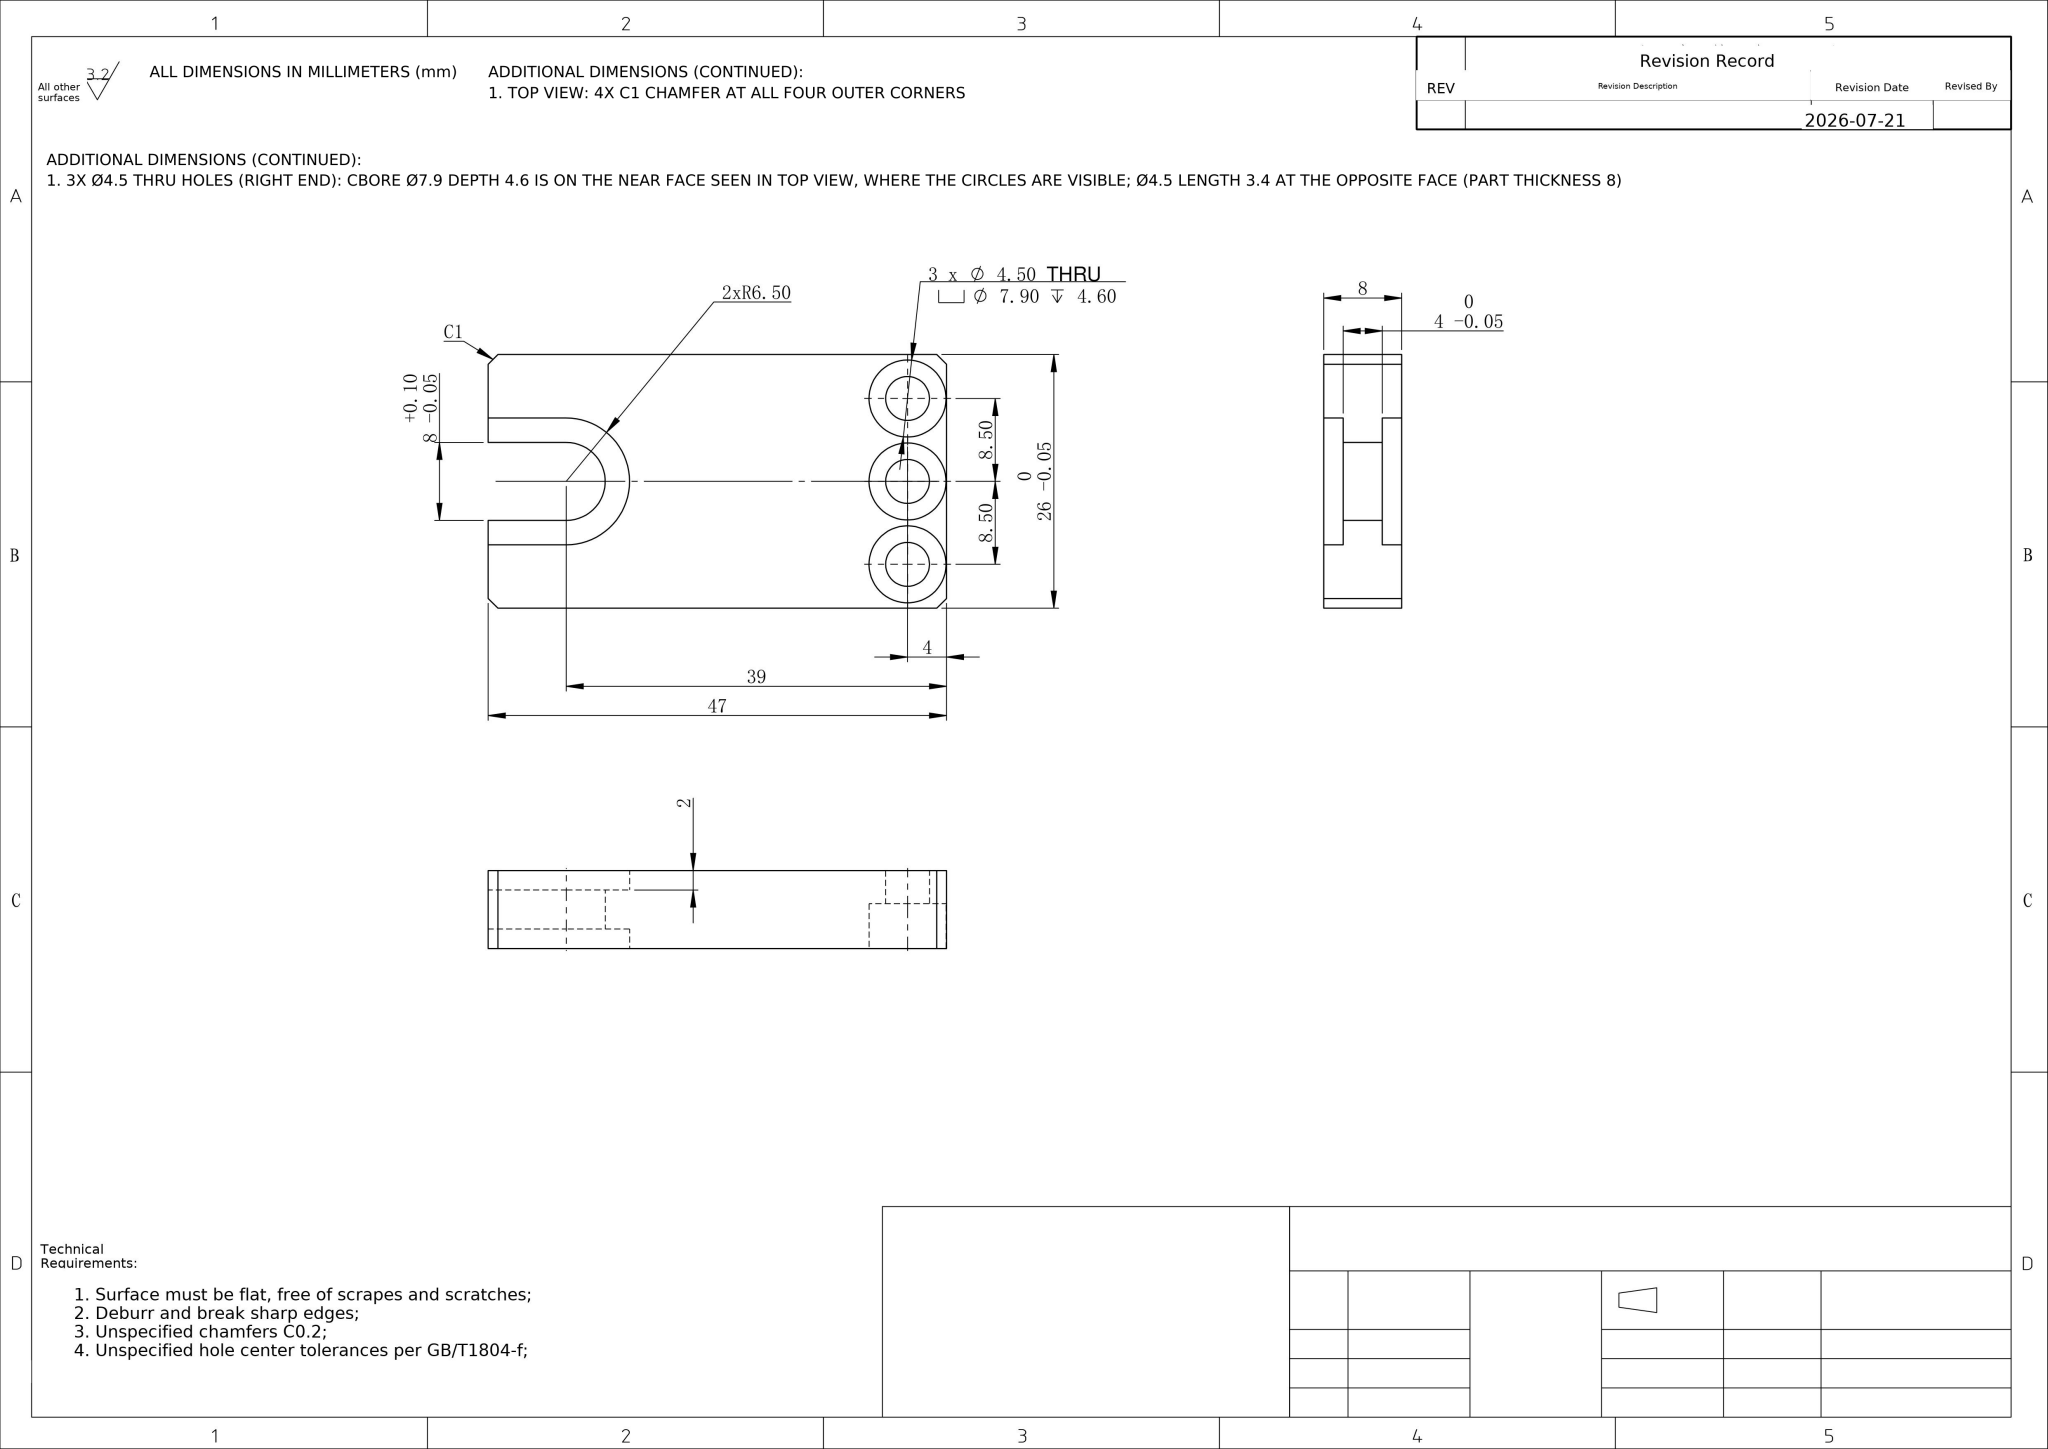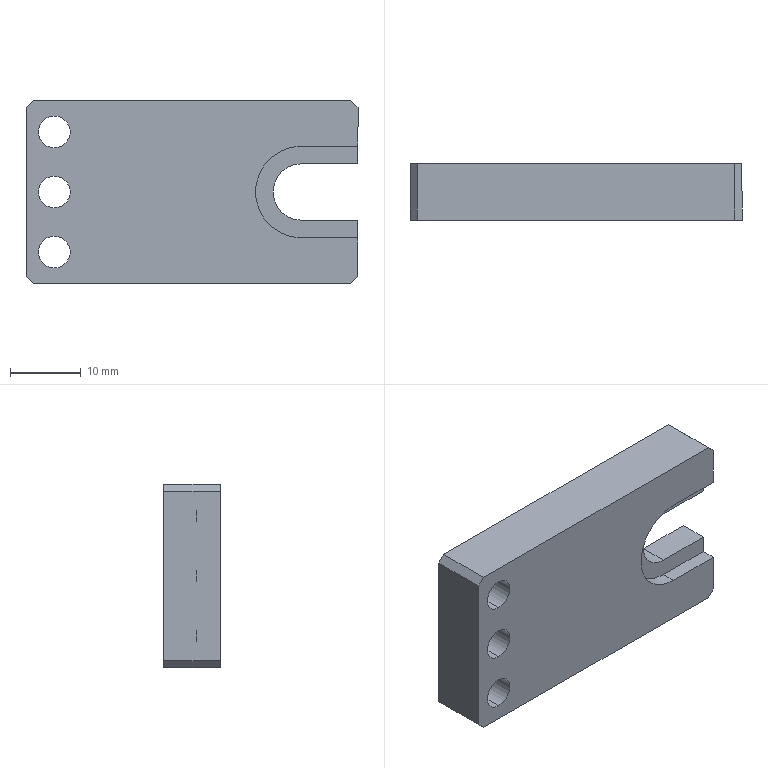Part | NX | mm | 1 solid | 37 faces | box 47 x 8 x 26 mm | volume 7883 mm3 | plane 22 | cylinder 15 | commonest cylinder face diameters 7.9 x6 4.5 x6 13 x2 8 x1